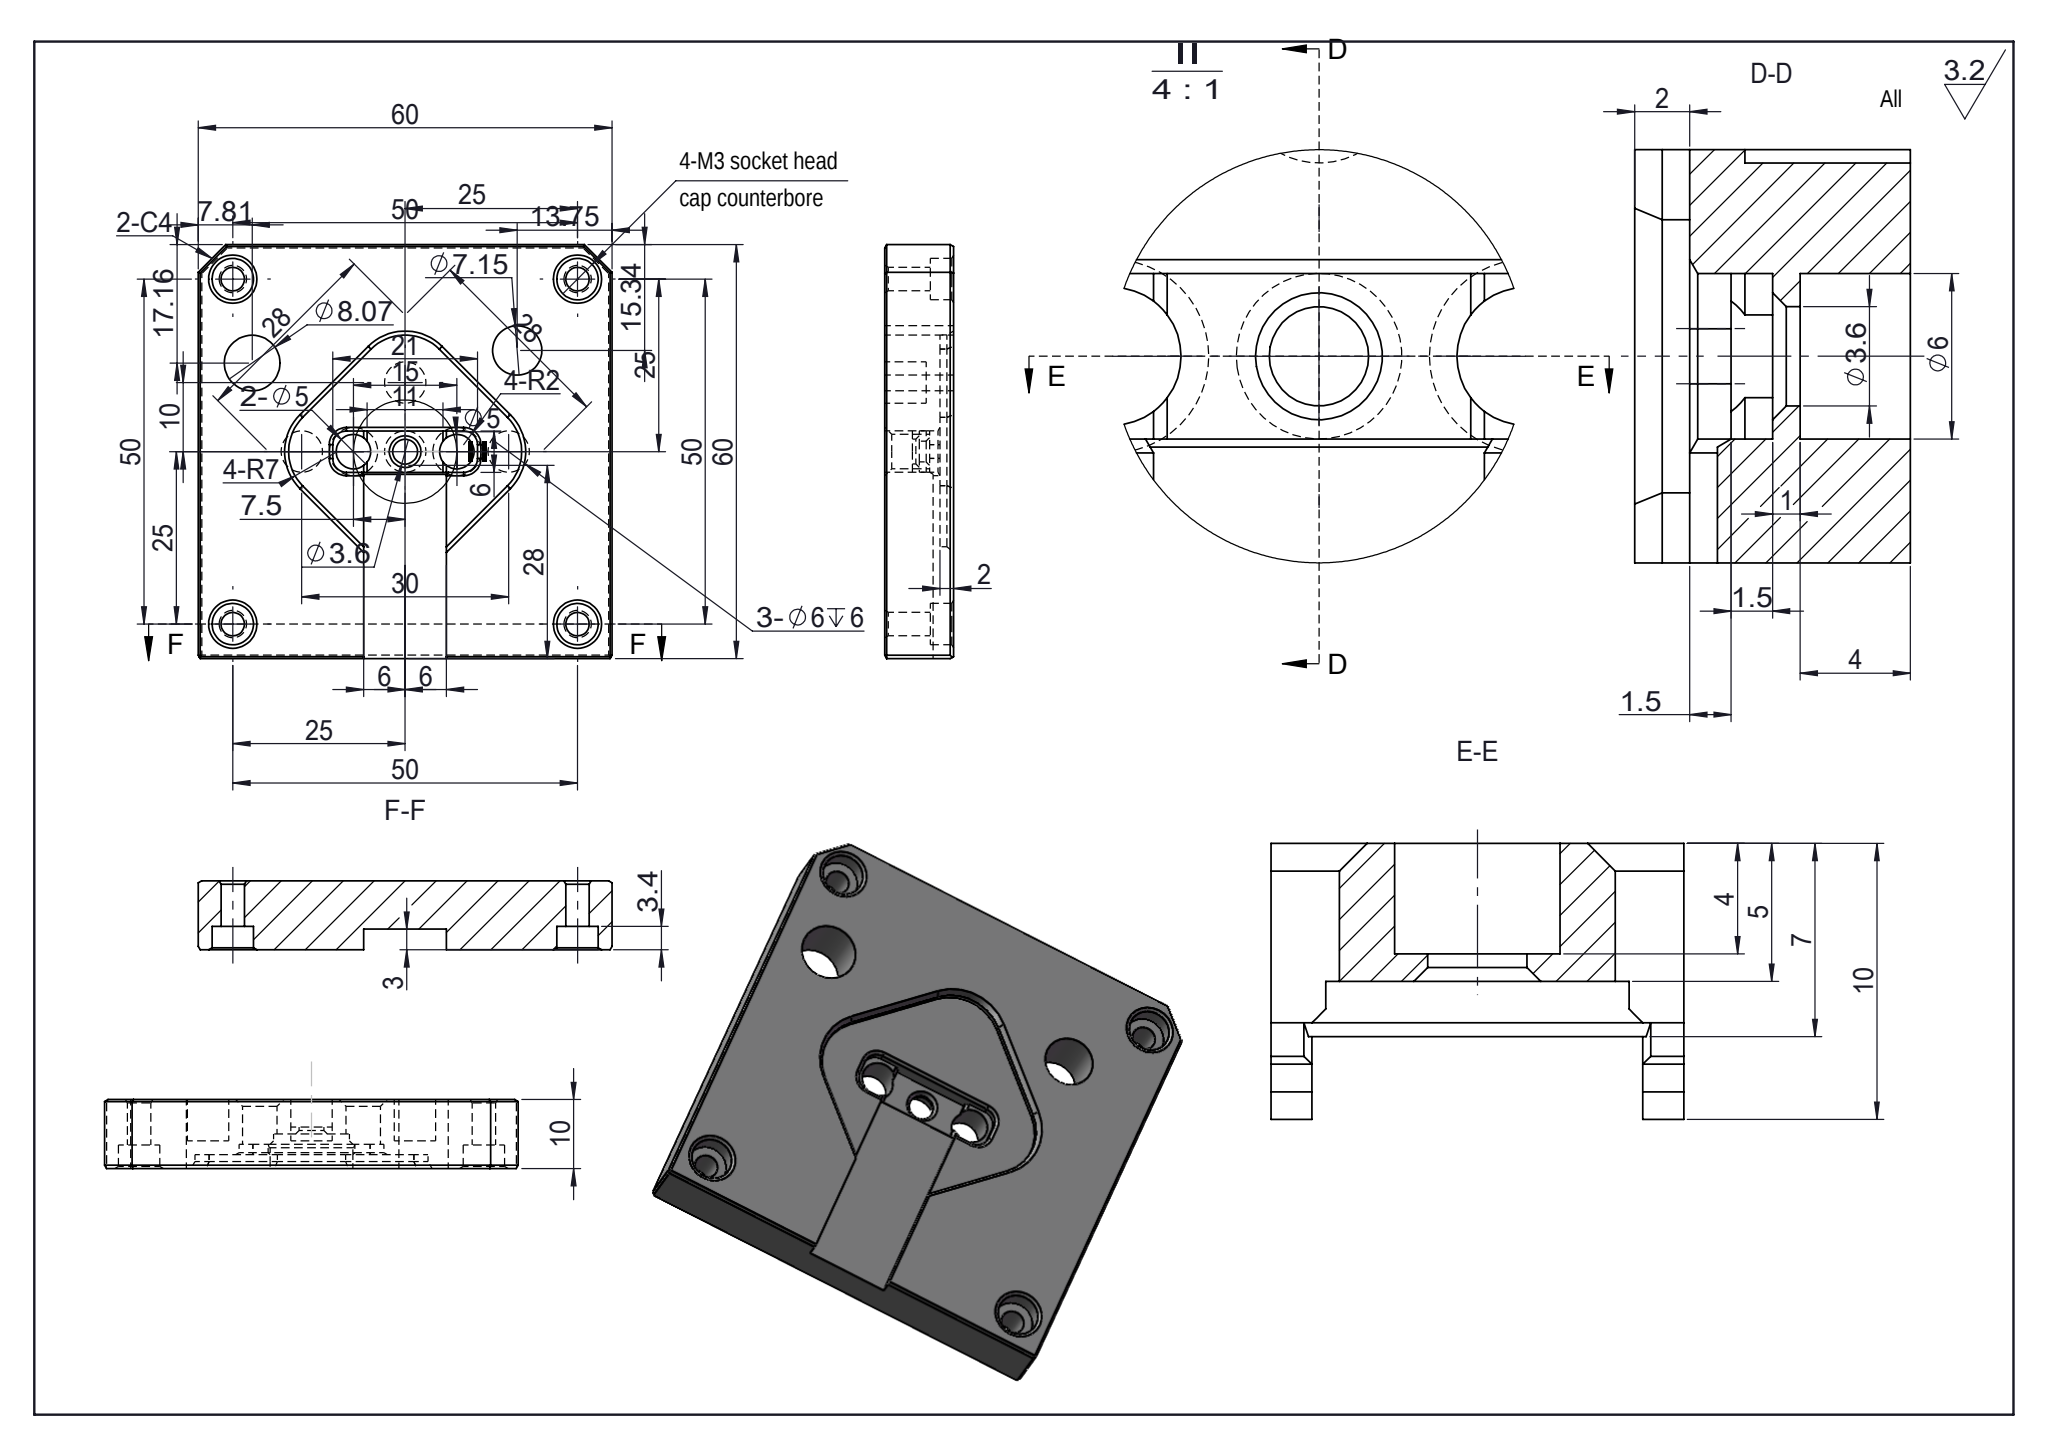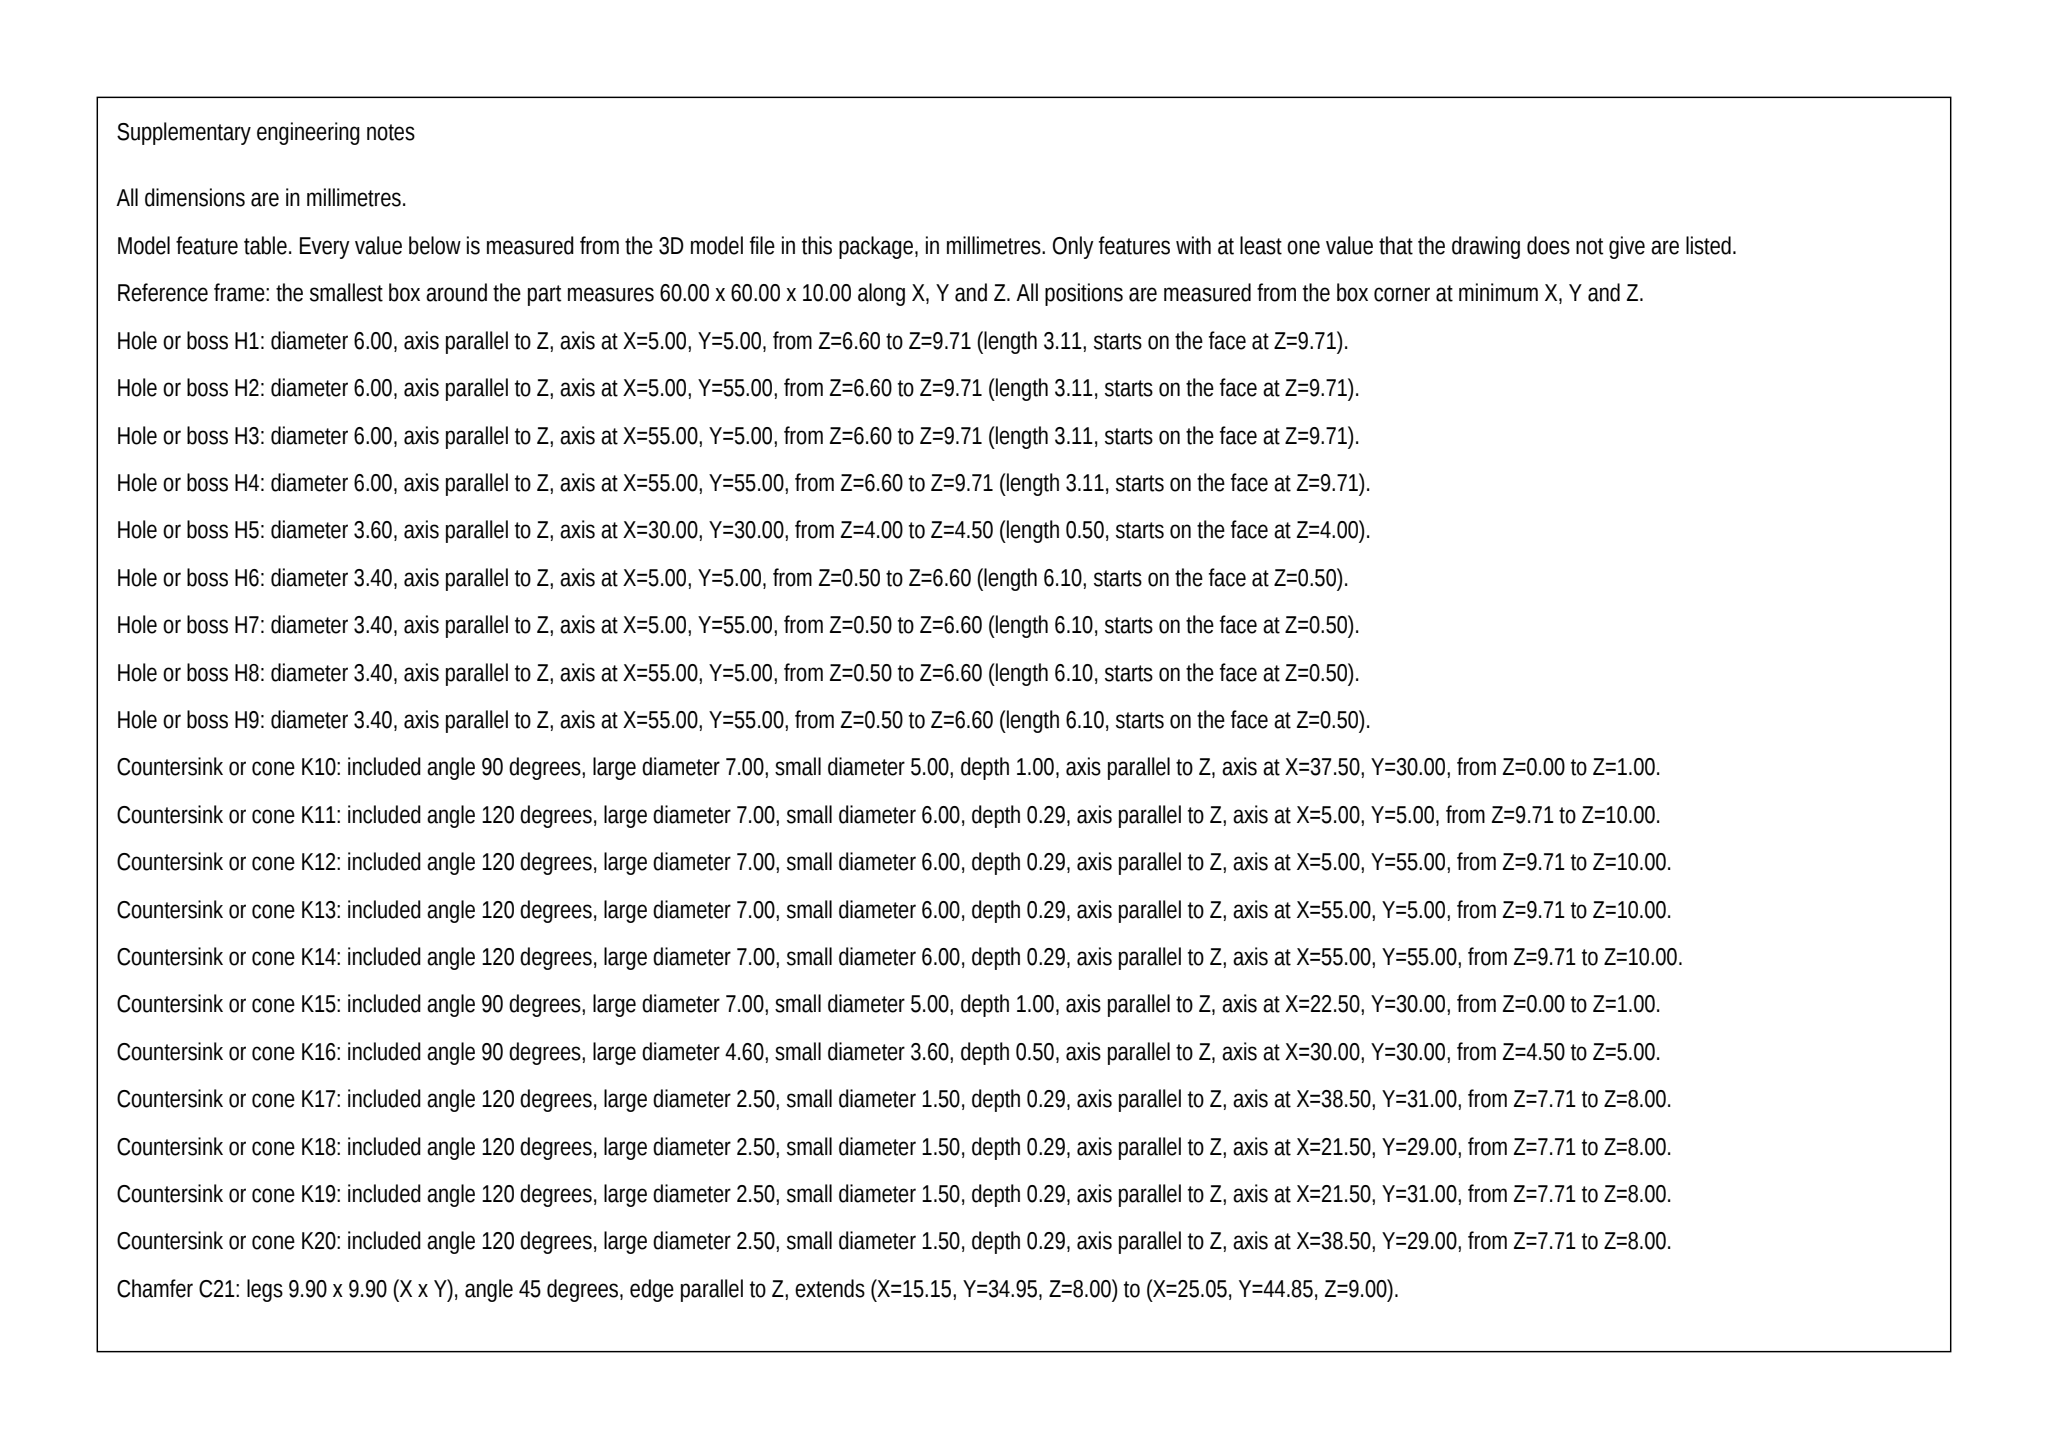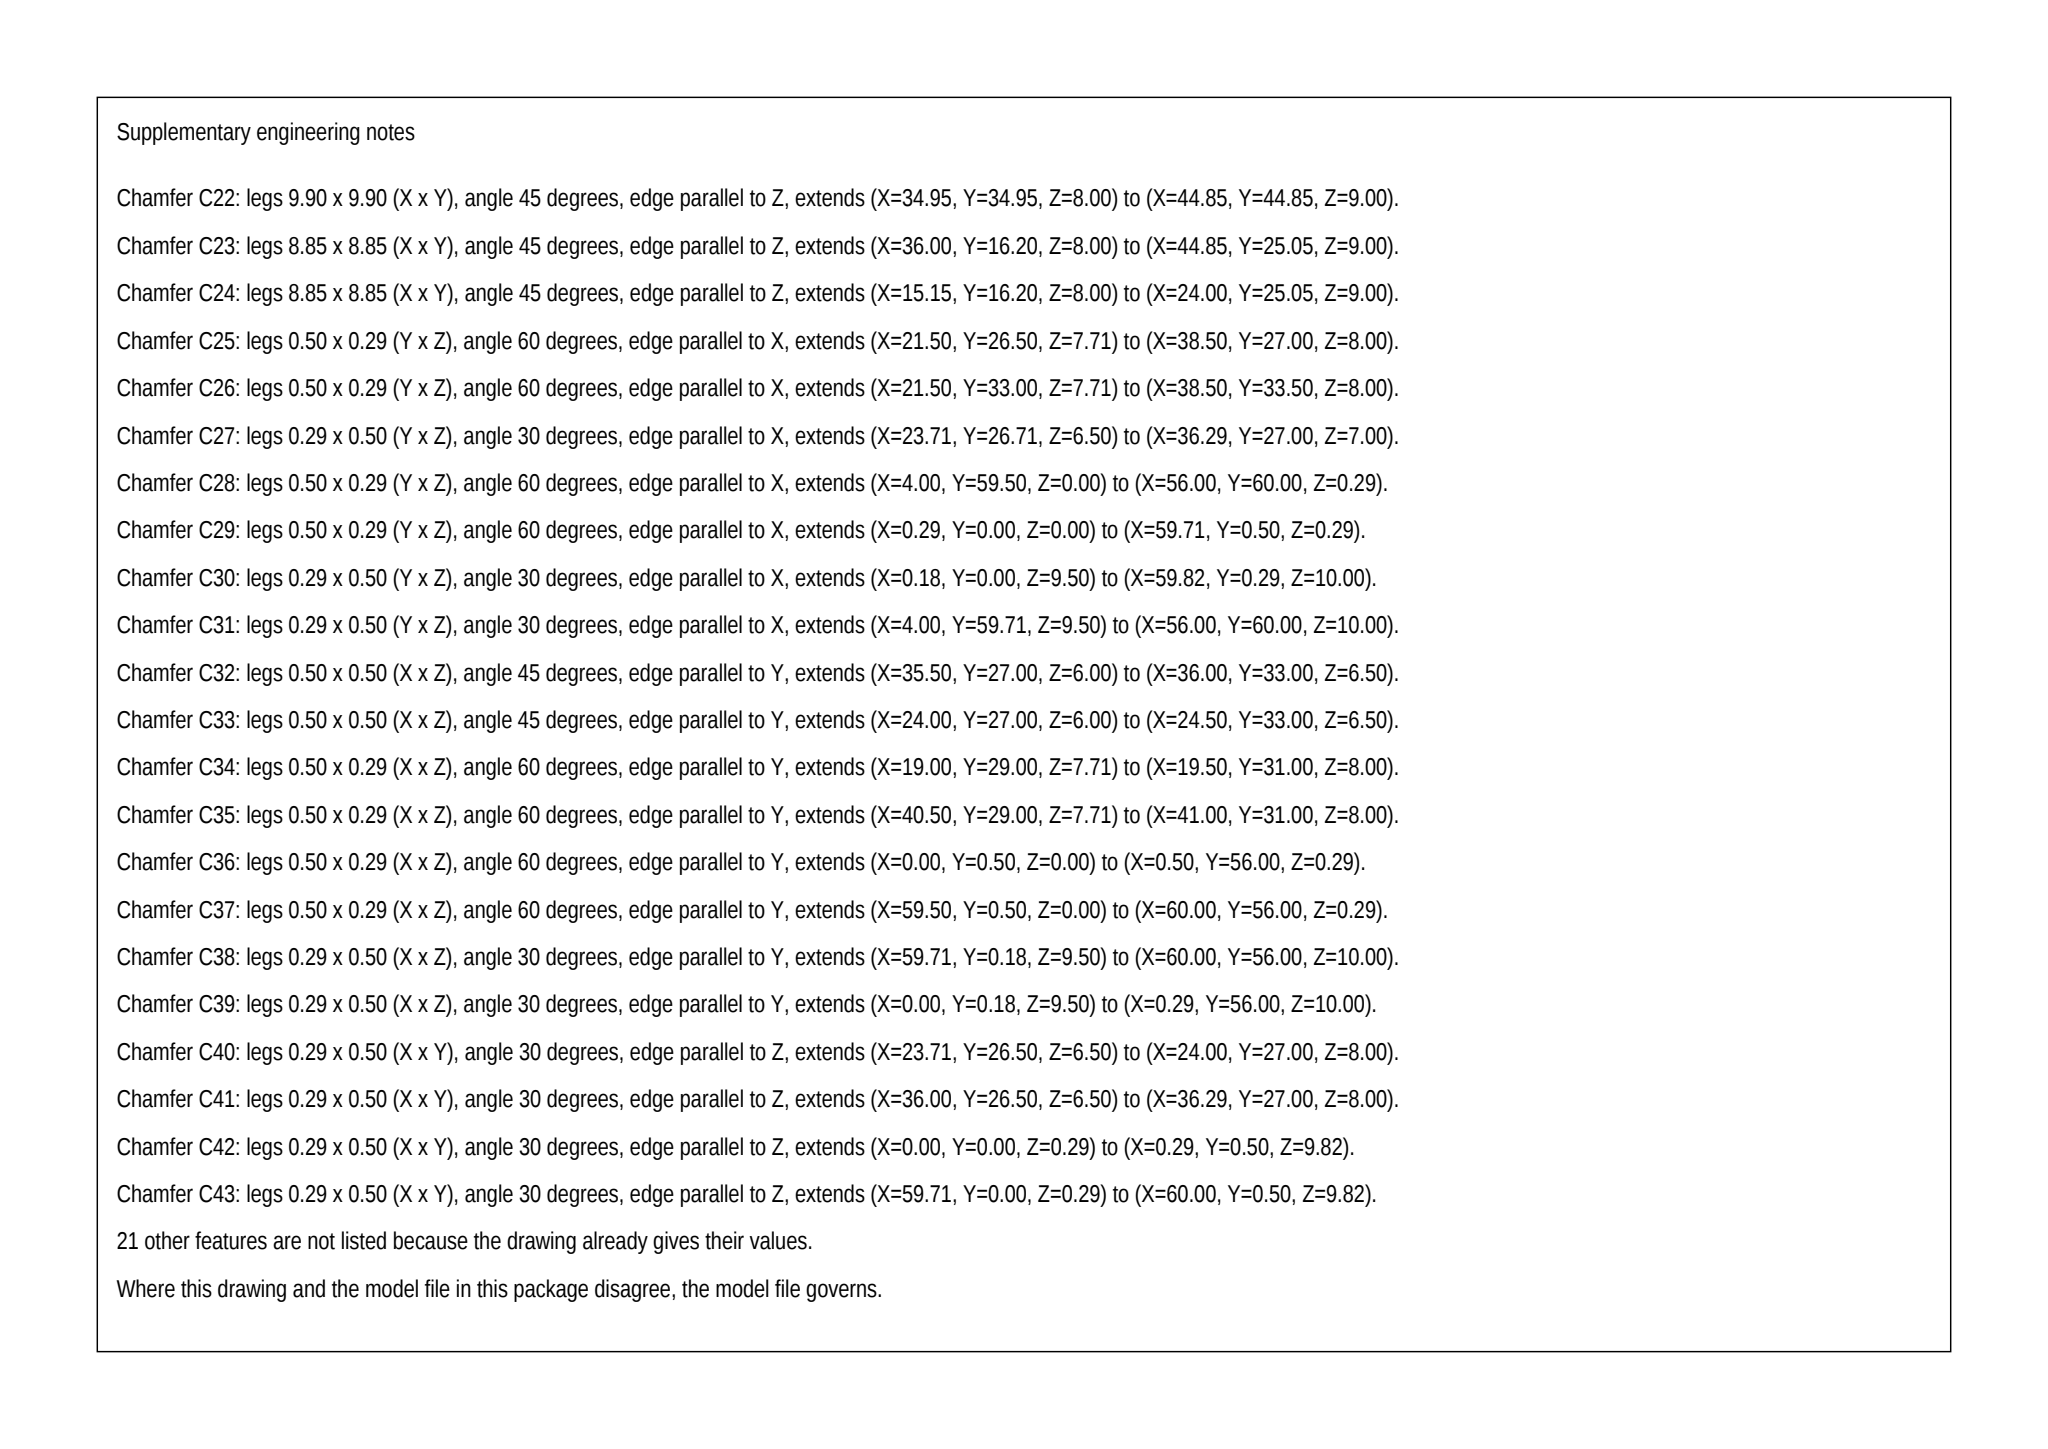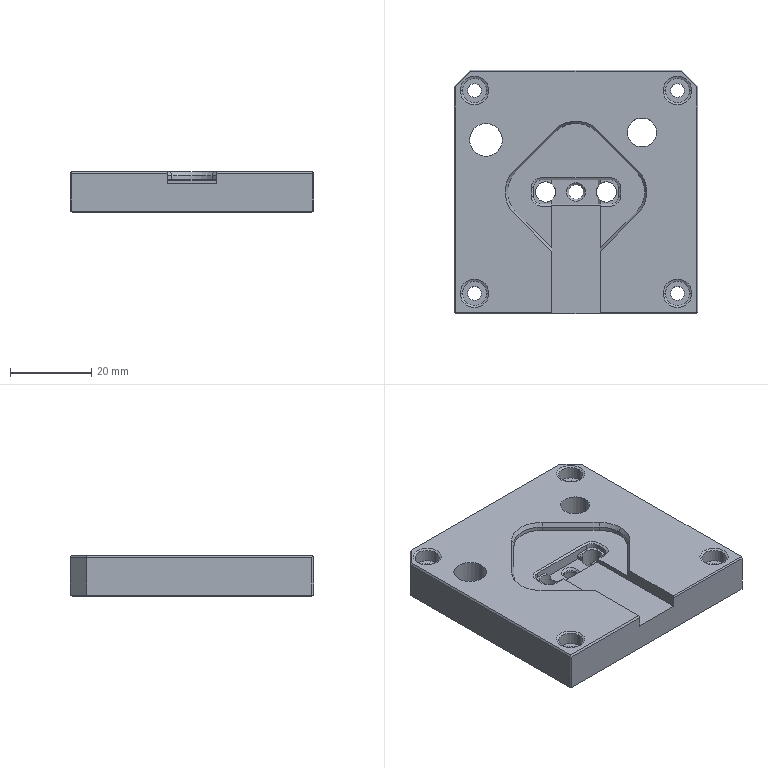Part | SolidWorks | mm | 1 solid | 142 faces | box 60 x 60 x 10 mm | volume 30897 mm3 | plane 70 | cylinder 42 | cone 30 | commonest cylinder face diameters 6 x16 3.4 x8 5 x4 14 x4 4 x4 8.072 x2 7.155 x2 3.6 x2